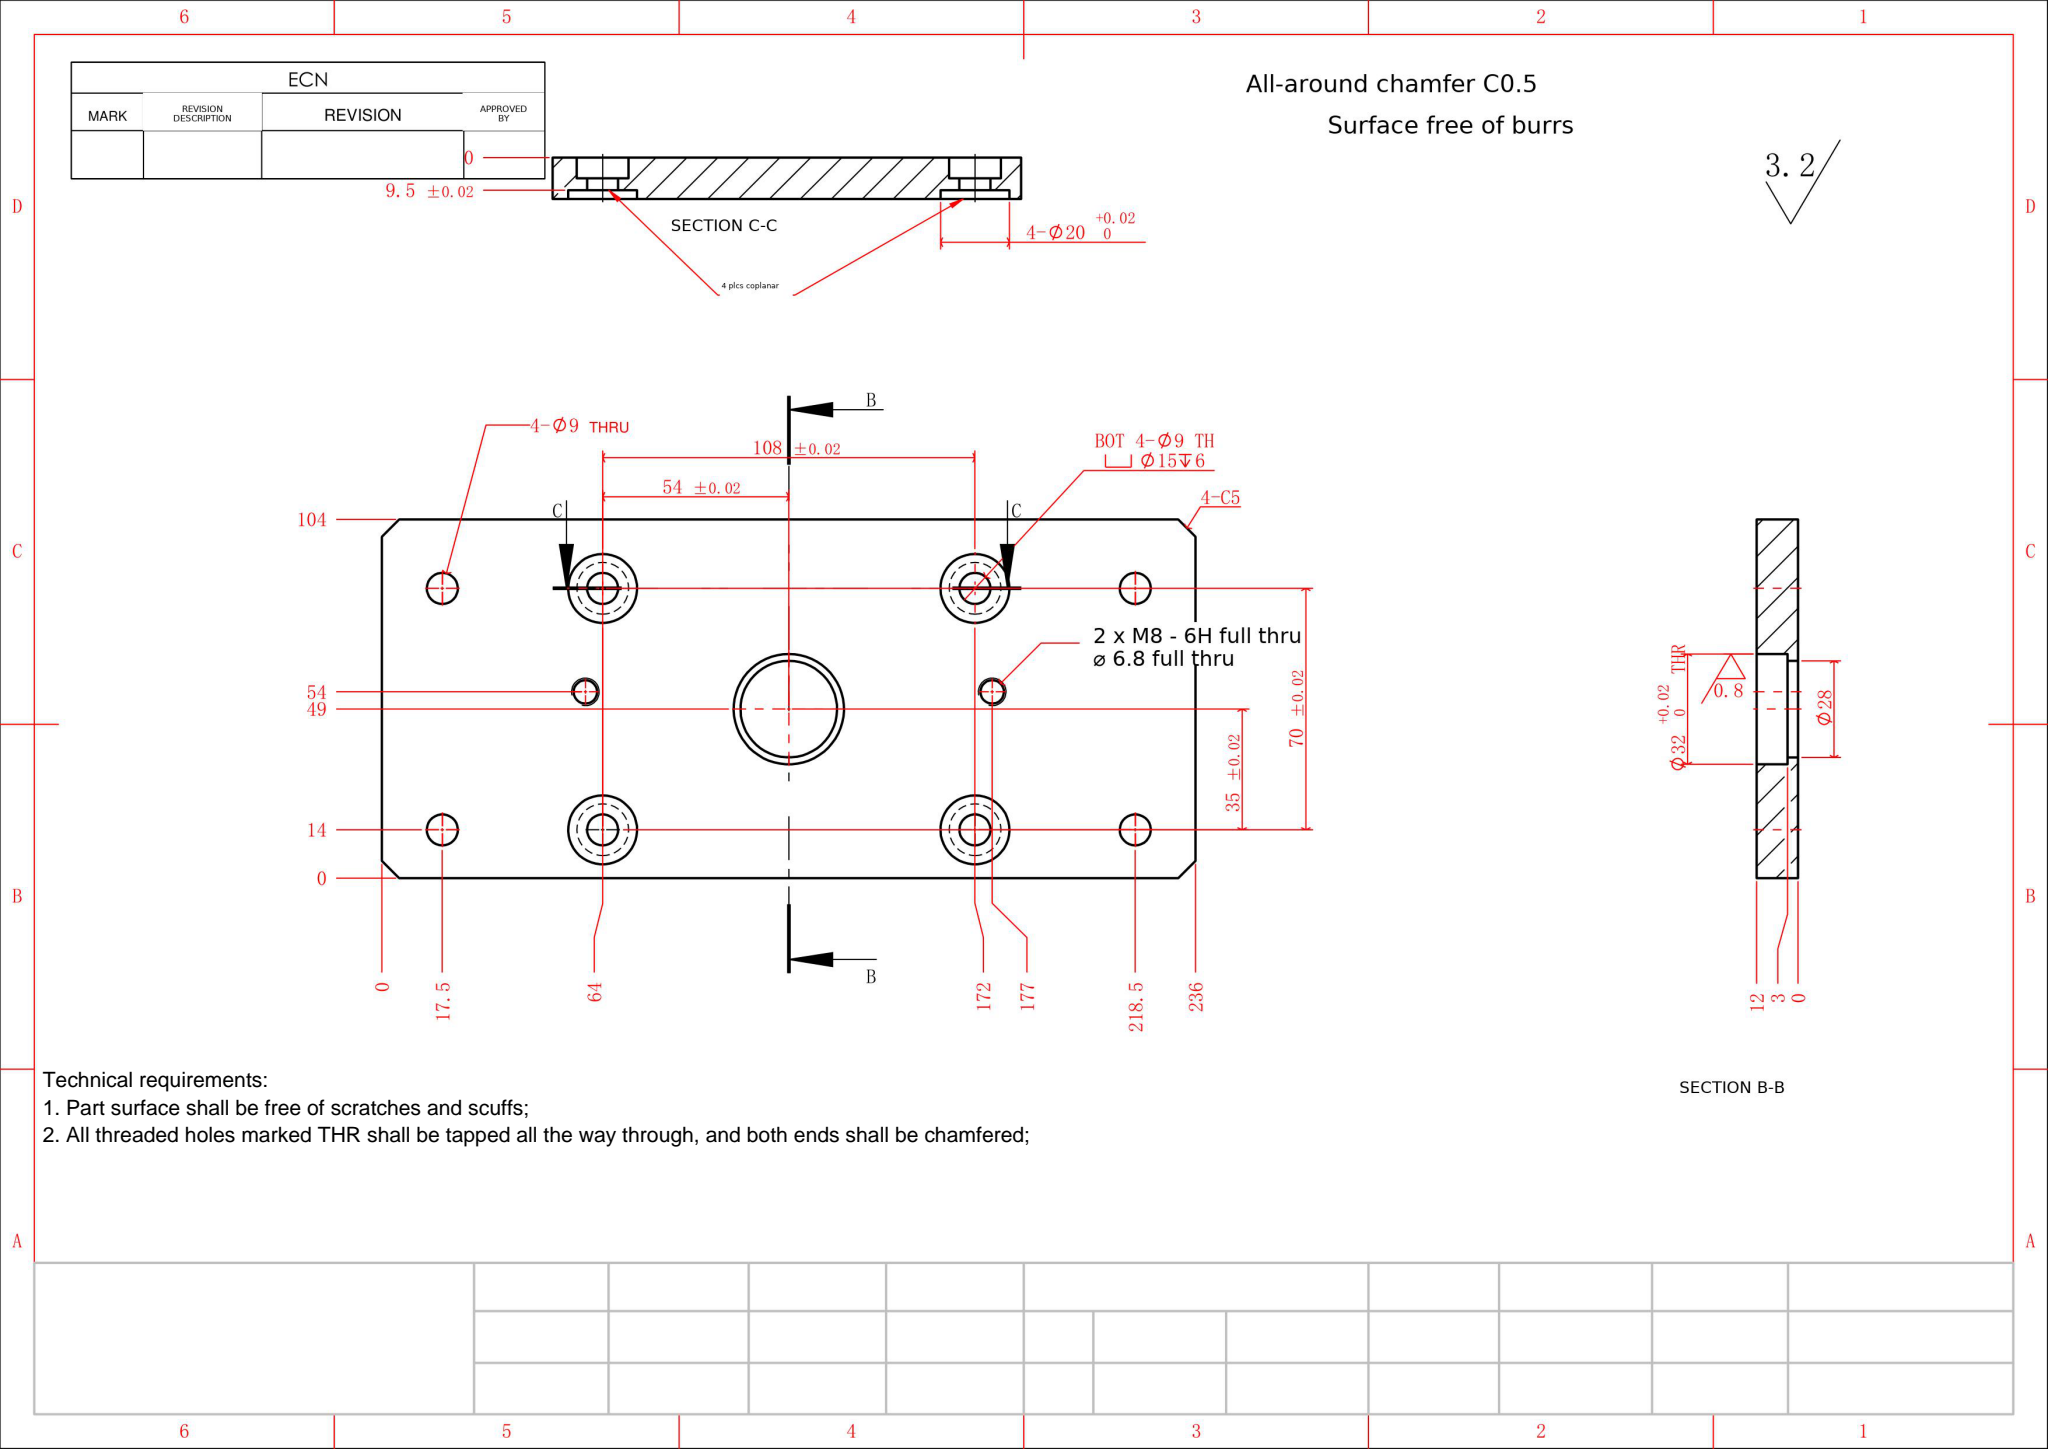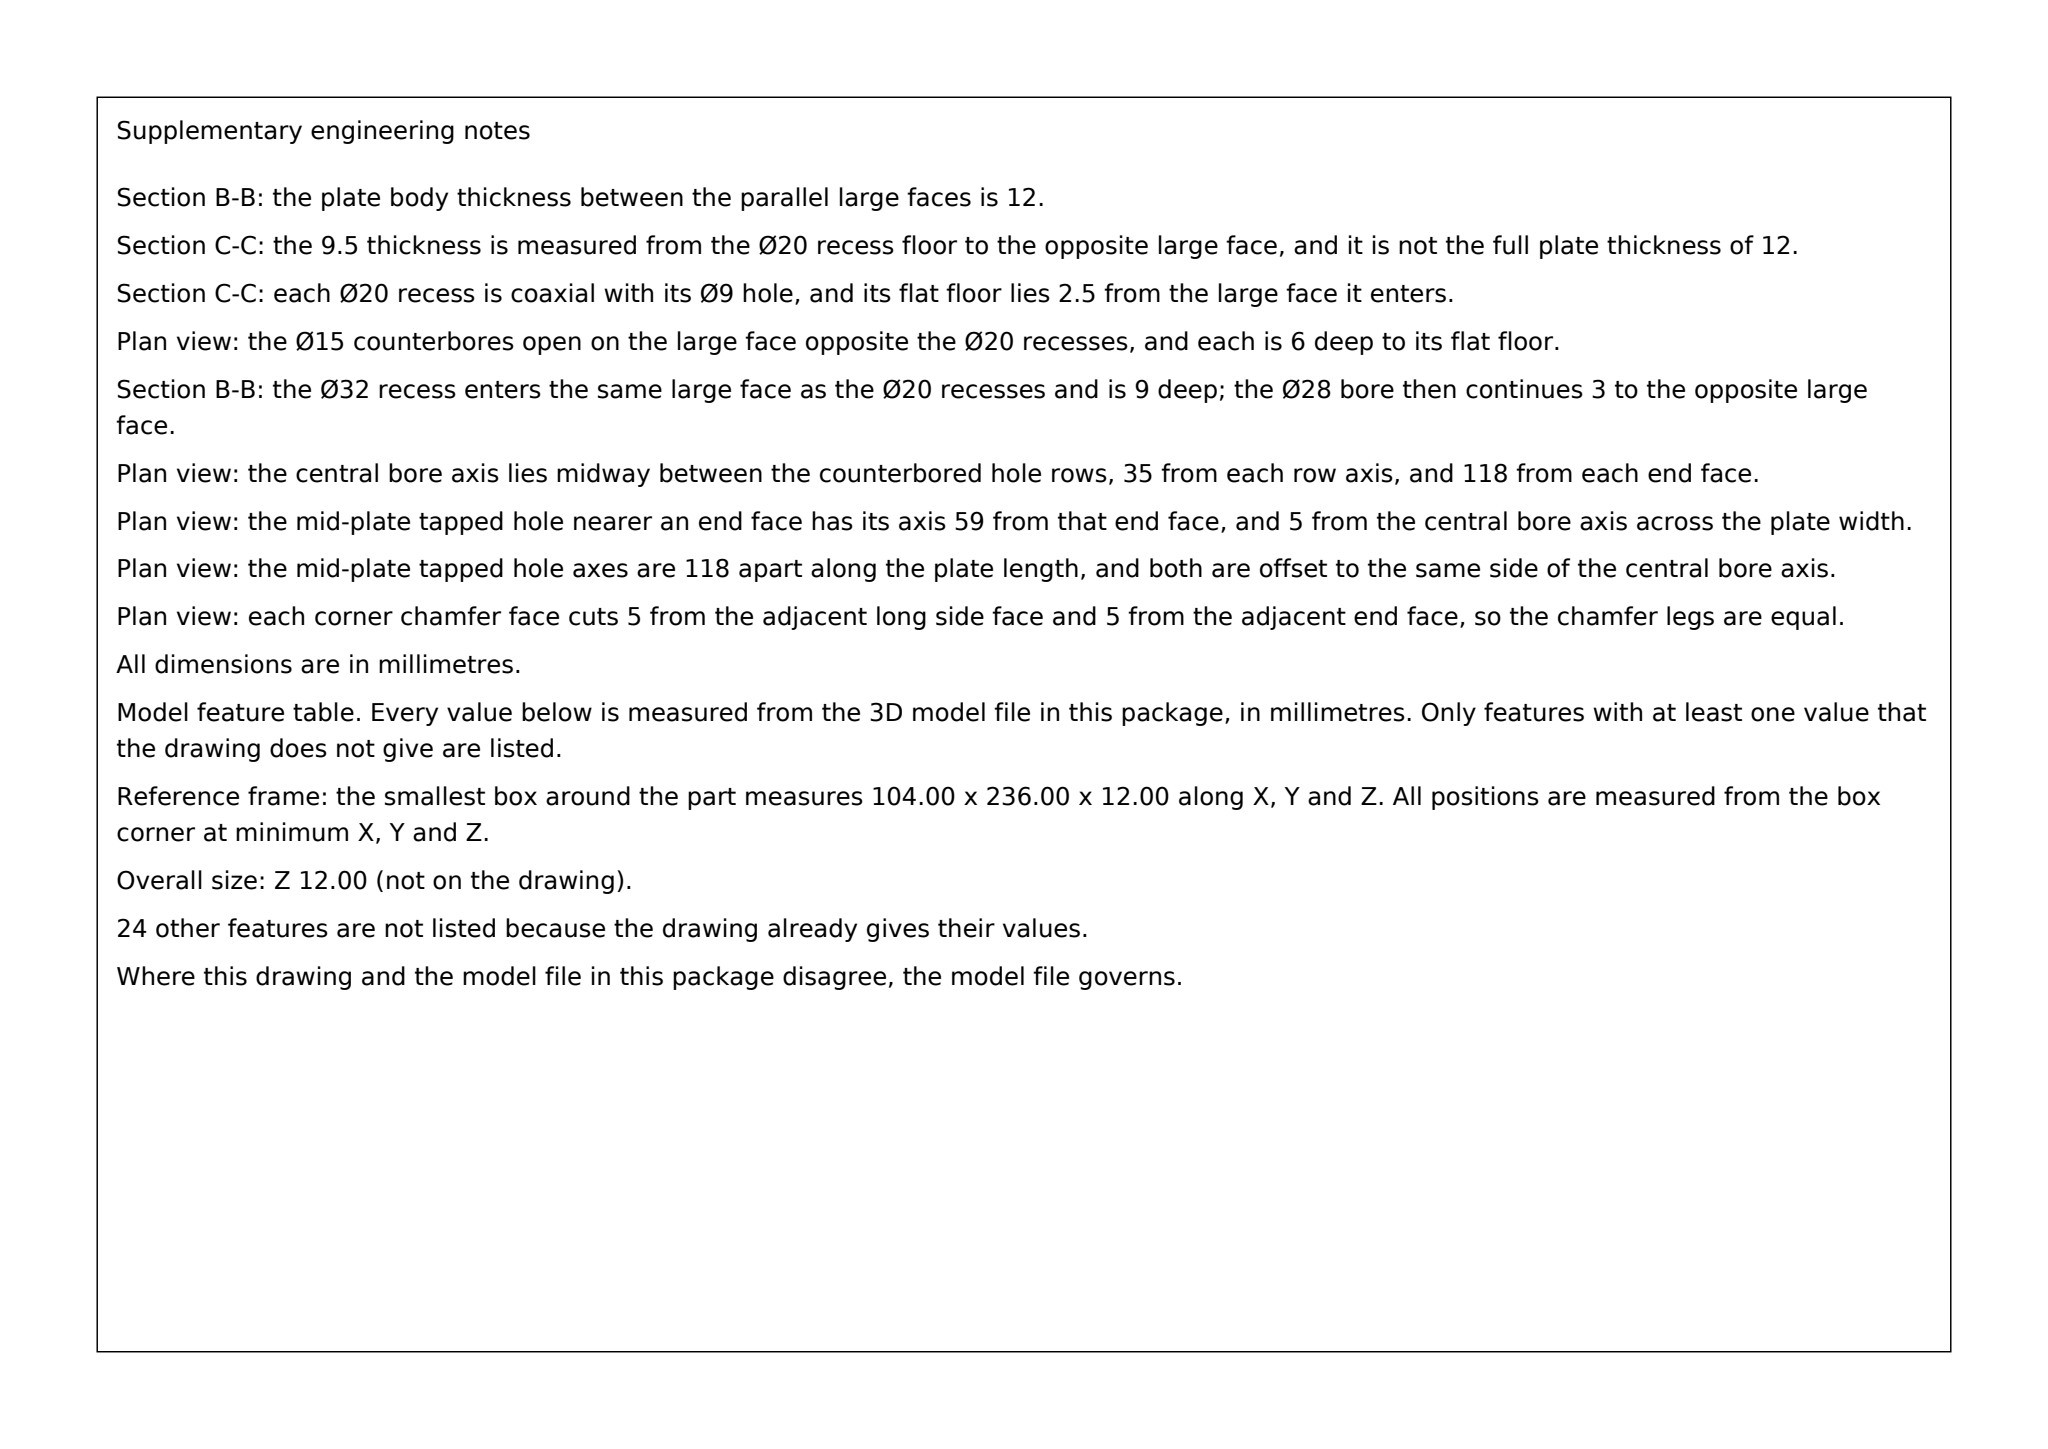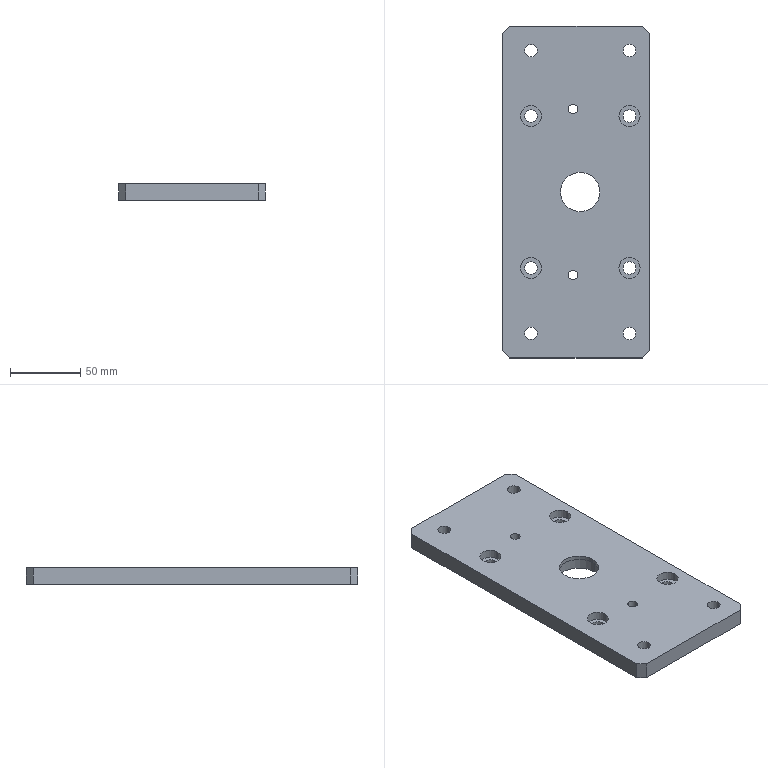Part | SolidWorks | mm | 1 solid | 59 faces | box 104 x 236 x 12 mm | volume 272644 mm3 | cylinder 40 | plane 19 | commonest cylinder face diameters 9 x16 15 x8 20 x8 6.8 x4 28 x2 32 x2
Drawing notes:
4-Ø20 CBORE DP 2.5 FROM BOT FACE; 9.5 TO CBORE FLOOR | from the solid: cyl Ø20 z-length 2.5 at z=0..2.5; plate thk 12; 12-2.5=9.5